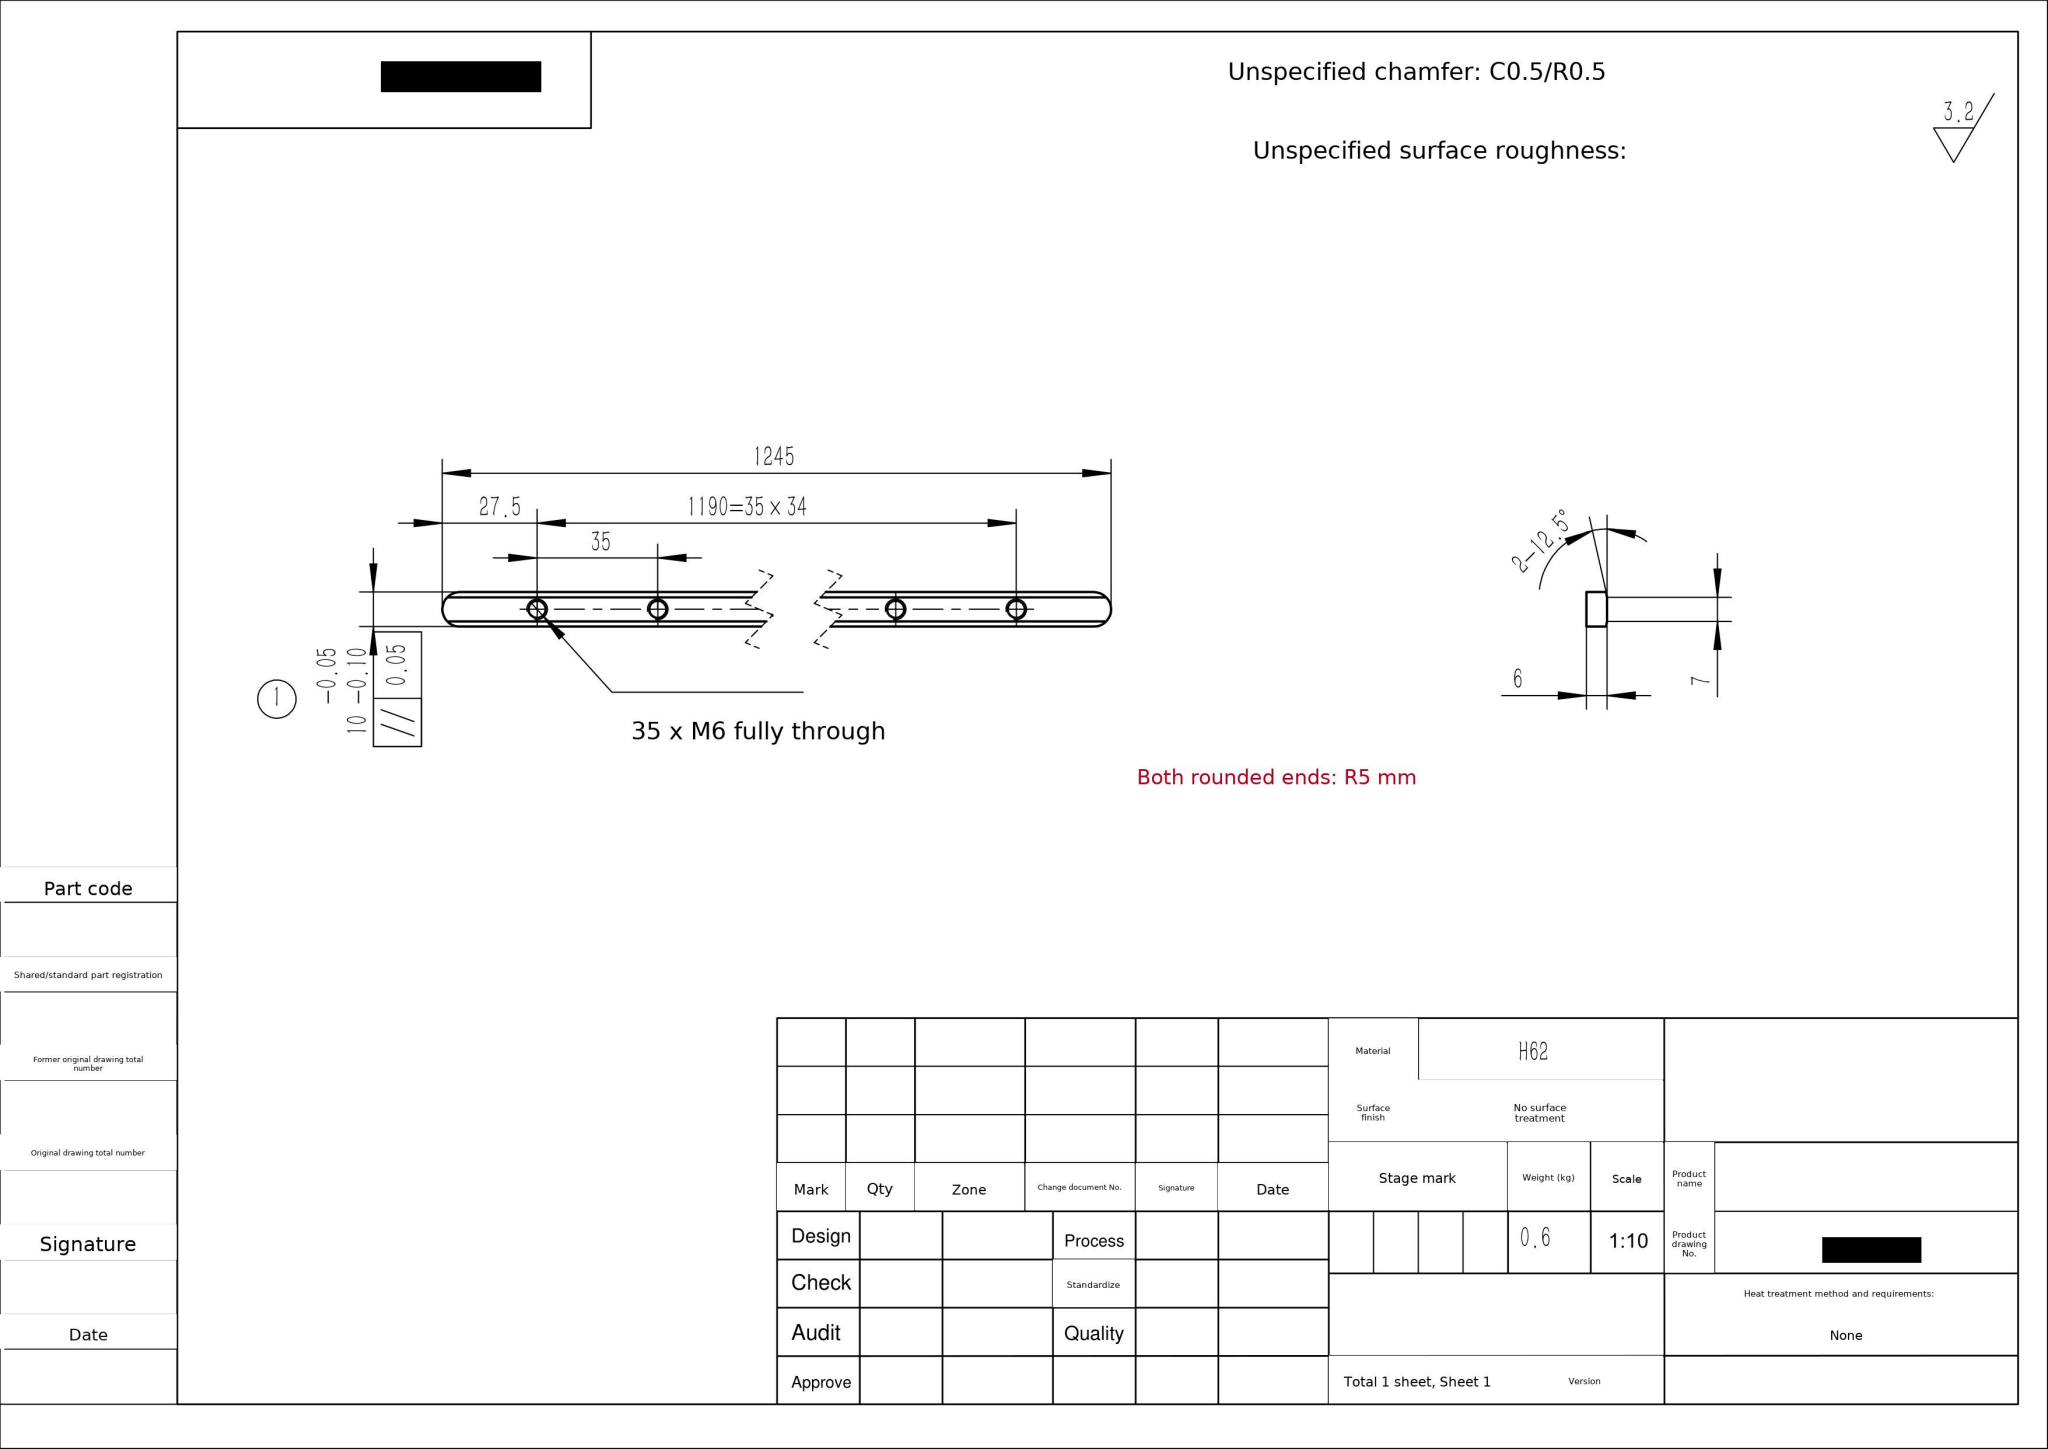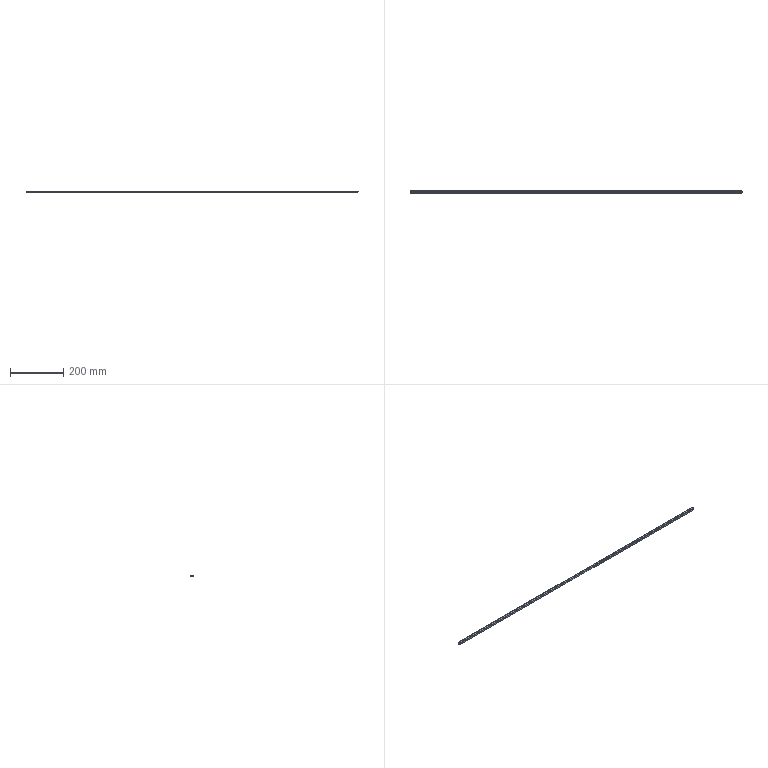Part | SolidWorks | mm | material H62 | 1 solid | 79 faces | box 1245 x 10 x 6 mm | volume 69830 mm3 | cylinder 73 | plane 6 | commonest cylinder face diameters 5 x70 10 x3
build123d program:
from build123d import *

# Parameters (mm, degrees)
BOSS_EXTRUDE1_DEPTH = 6
M6_TAPPED_HOLE2_D   = 5
LPATTERN2_COUNT     = 18
LPATTERN2_PITCH     = 35
LPATTERN3_COUNT     = 18
LPATTERN3_PITCH     = 35
CUT_EXTRUDE4_DEPTH  = 1246.024


with BuildPart() as part:
    # Sketch1 → Boss-Extrude1 (new body)
    with BuildSketch(Plane.XY):
        with BuildLine():
            Line((0, 5), (1235, 5))
            ThreePointArc((1235, 5), (1240, 0), (1235, -5))
            Line((1235, -5), (0, -5))
            ThreePointArc((0, -5), (-5, 0), (0, 5))
        make_face()
    extrude(amount=BOSS_EXTRUDE1_DEPTH)

    # M6 Tapped Hole2 (through all)
    with Locations(Plane.XY.offset(6)):
        with Locations((617.5, 0)):
            m6_tapped_hole2 = Hole(M6_TAPPED_HOLE2_D / 2)

    # LPattern2: M6 Tapped Hole2 ×18
    with Locations(*[(i * LPATTERN2_PITCH, 0, 0) for i in range(1, LPATTERN2_COUNT)]):
        add(m6_tapped_hole2, mode=Mode.SUBTRACT)

    # LPattern3: M6 Tapped Hole2 ×18
    with Locations(*[(-i * LPATTERN3_PITCH, 0, 0) for i in range(1, LPATTERN3_COUNT)]):
        add(m6_tapped_hole2, mode=Mode.SUBTRACT)

    # Sketch8 → Cut-Extrude4 (cut, through all)
    with BuildSketch(Plane.ZY.offset(5)):
        Polygon((6, 3.5), (6, 8.24), (4.949, 8.24), align=None)
        Polygon((6, -8.24), (4.949, -8.24), (6, -3.5), align=None)
    extrude(amount=-CUT_EXTRUDE4_DEPTH, mode=Mode.SUBTRACT)


solid = part.part